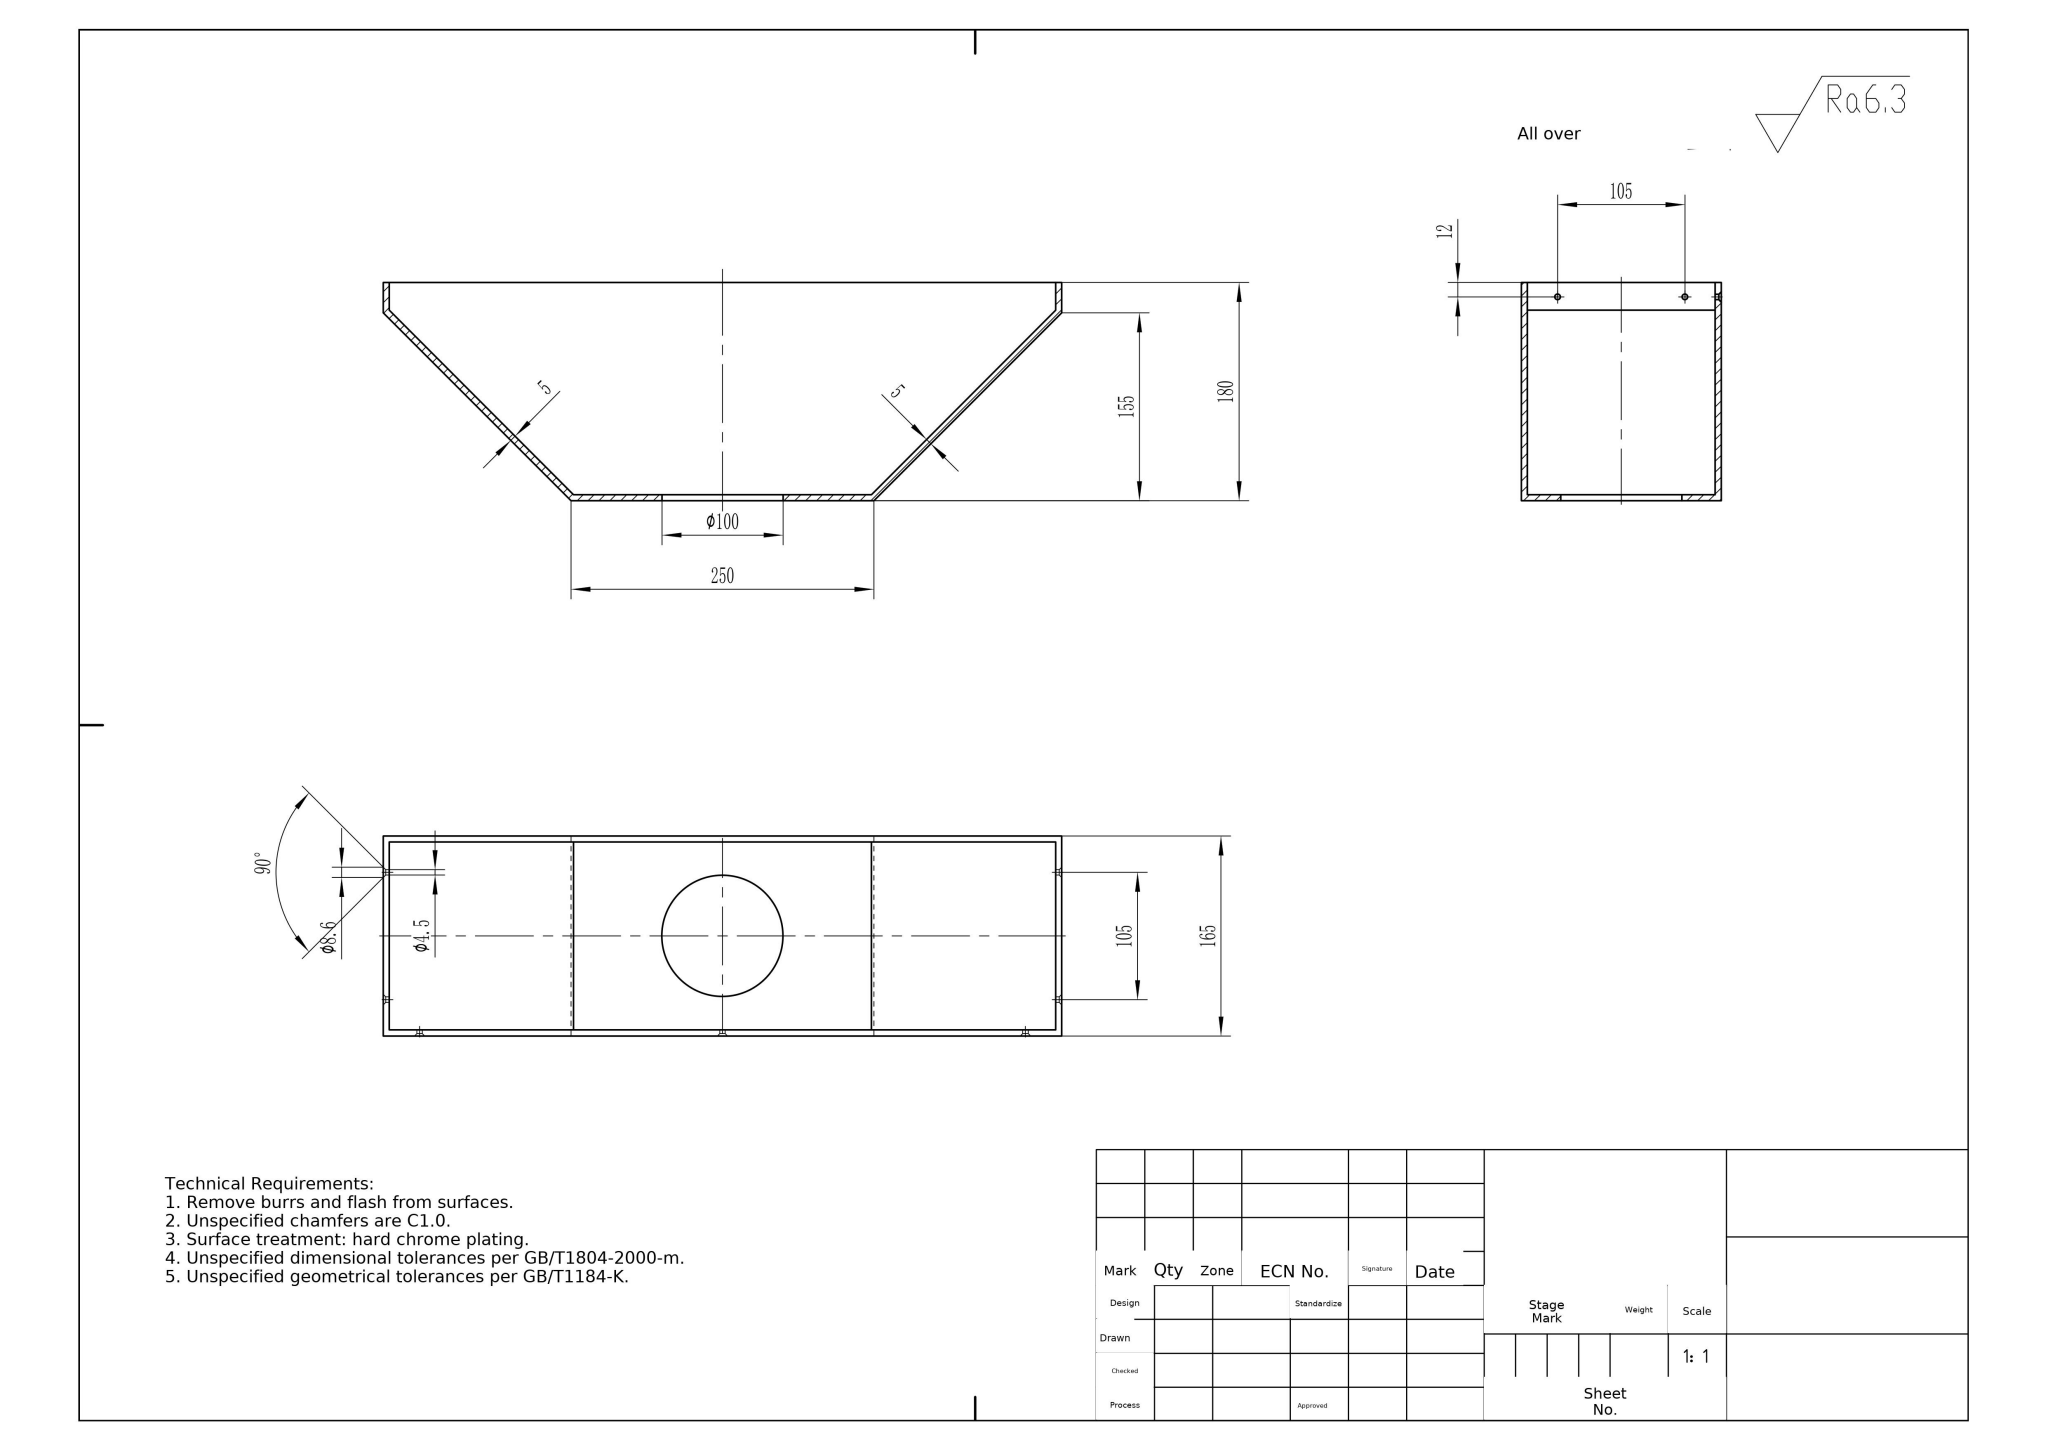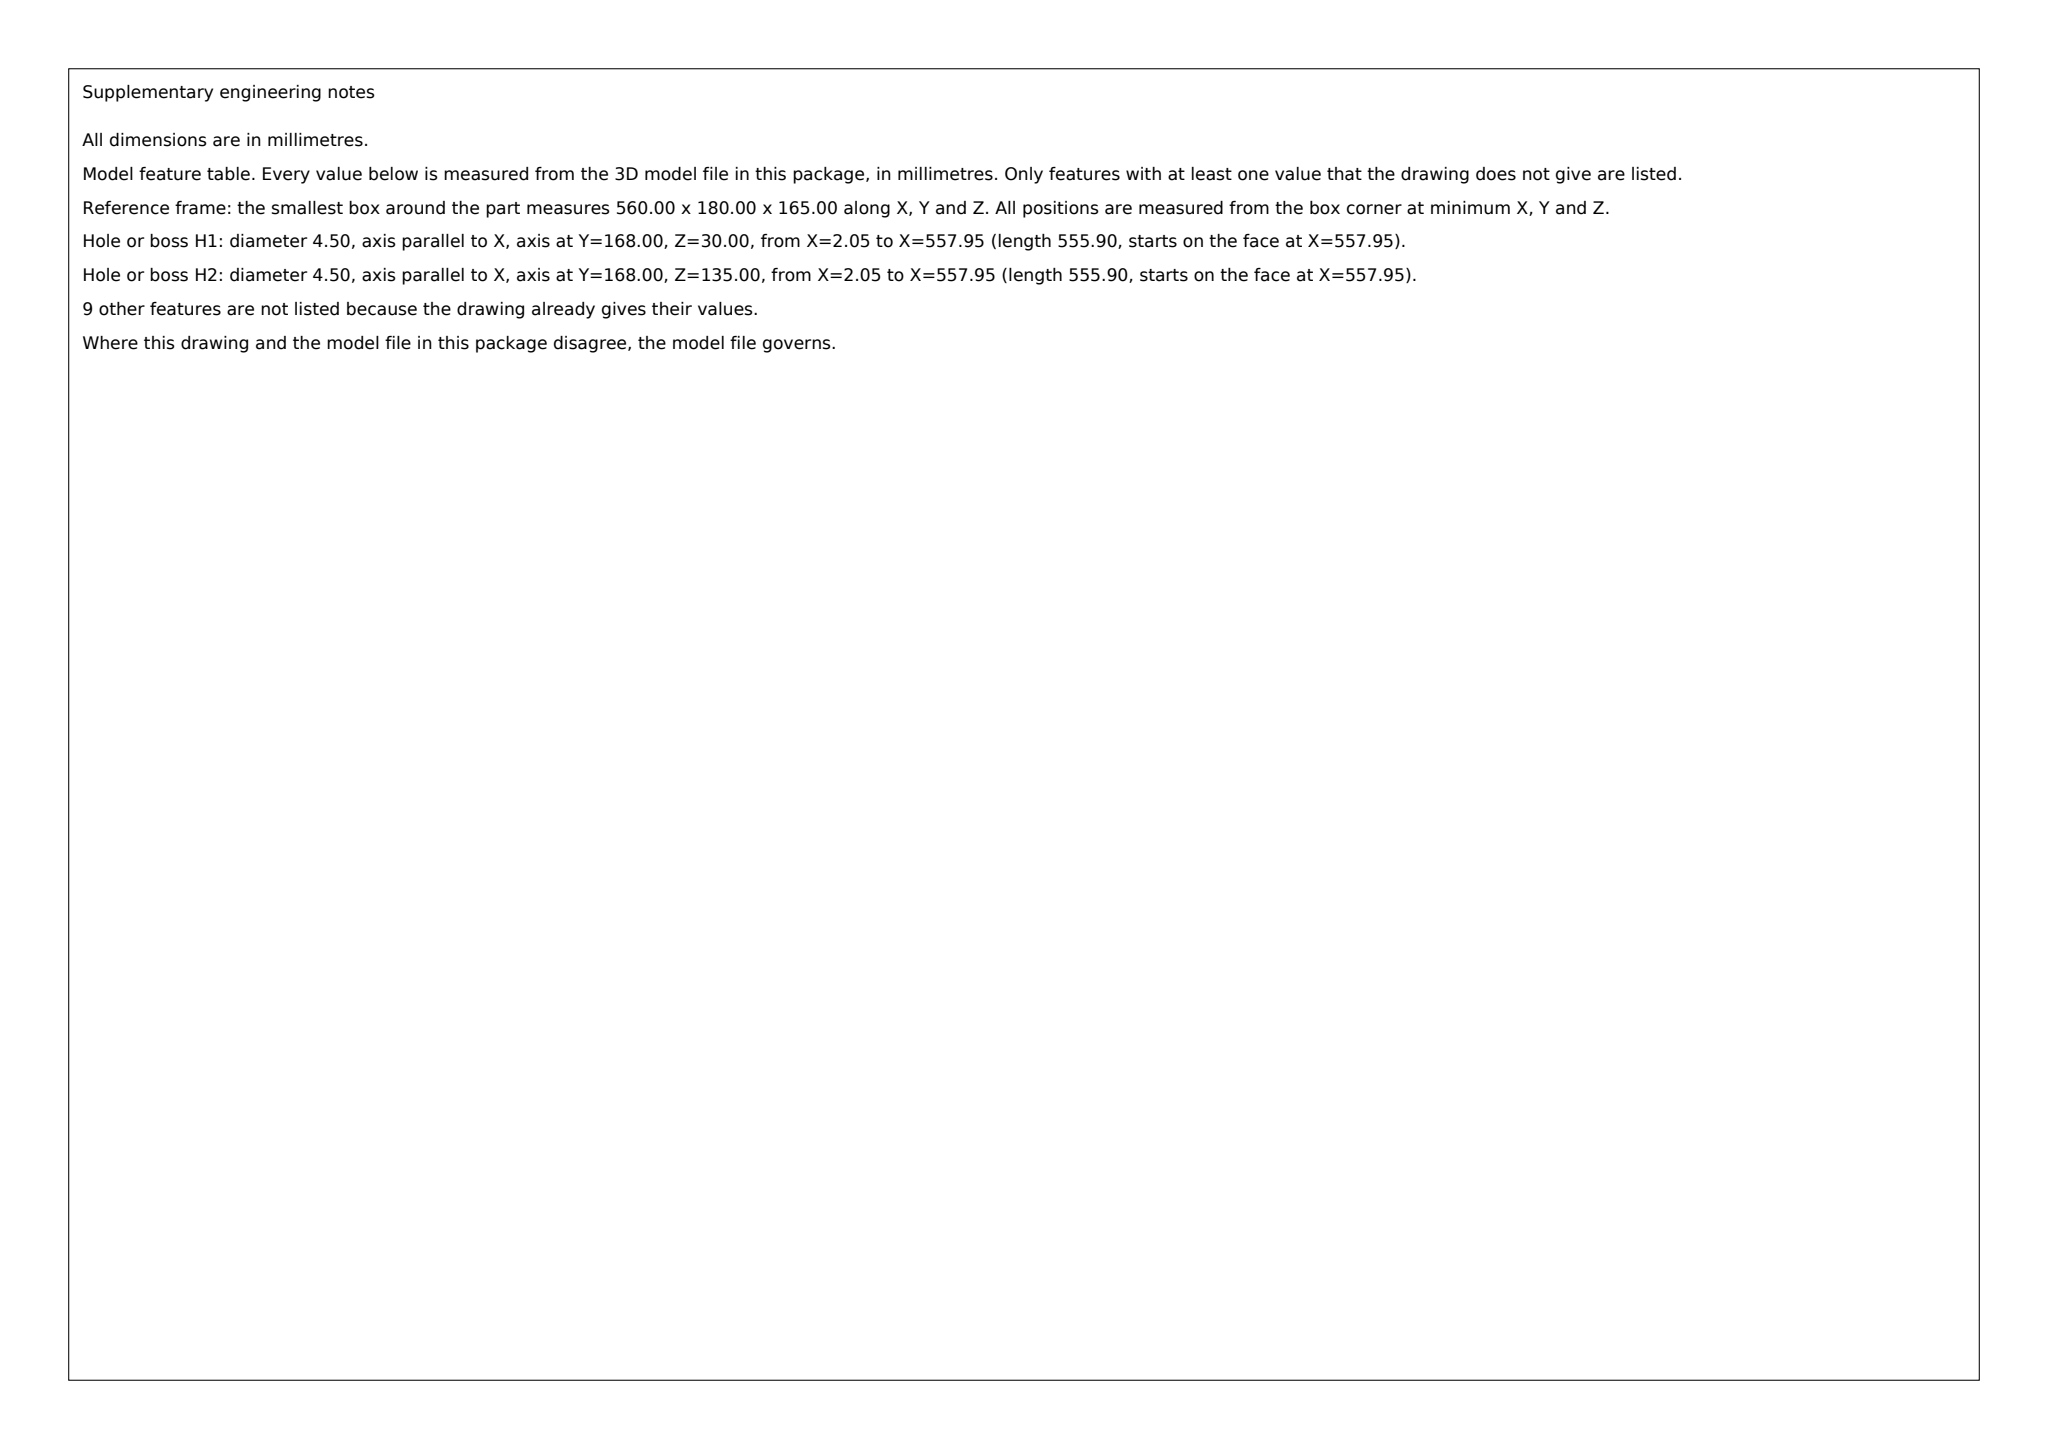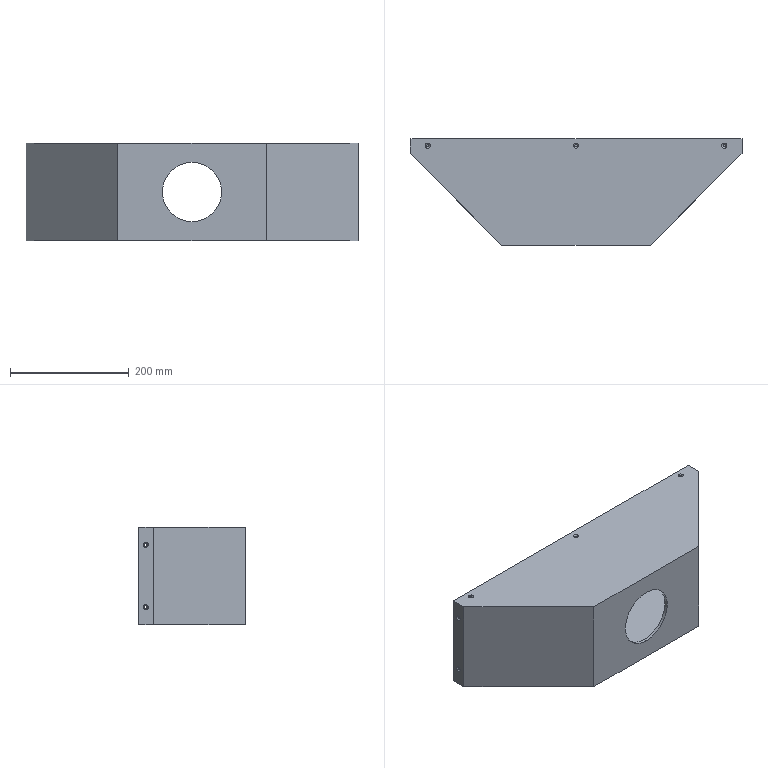Part | SolidWorks | mm | 1 solid | 45 faces | box 560 x 180 x 165 mm | volume 1293497 mm3 | cylinder 16 | plane 15 | cone 14 | commonest cylinder face diameters 4.5 x14 100 x2
build123d program:
from build123d import *

# Parameters (mm, degrees)
BOSS_EXTRUDE1_DEPTH                               = 82.5
SHELL1_T                                          = -5
SKETCH2_R                                         = 50
CUT_EXTRUDE1_DEPTH                                = 341.34
HOLE_SIZE_ACCORDING_TO_PHILLIPS_RAISE_D           = 4.5
HOLE_SIZE_ACCORDING_TO_PHILLIPS_RAISE_DEPTH       = 5.001
HOLE_SIZE_ACCORDING_TO_PHILLIPS_RAISE_CSINK_D     = 8.6
HOLE_SIZE_ACCORDING_TO_PHILLIPS_RAISE_CSINK_ANGLE = 90
MIRROR2_COPY_1_D                                  = 4.5
MIRROR2_COPY_1_DEPTH                              = 5.001
MIRROR2_COPY_1_CSINK_D                            = 8.6
MIRROR2_COPY_1_CSINK_ANGLE                        = 90
HOLE_SIZE_ACCORDING_TO_PHILLIPS_R_2_D             = 4.5
HOLE_SIZE_ACCORDING_TO_PHILLIPS_R_2_DEPTH         = 5
HOLE_SIZE_ACCORDING_TO_PHILLIPS_R_2_CSINK_D       = 8.6
HOLE_SIZE_ACCORDING_TO_PHILLIPS_R_2_CSINK_ANGLE   = 90


with BuildPart() as part:
    # Sketch1 → Boss-Extrude1 (new, symmetric)
    with BuildSketch(Plane.XY):
        Polygon((125, 0), (-125, 0), (-280, 155), (-280, 180), (280, 180), (280, 155), align=None)
    extrude(amount=BOSS_EXTRUDE1_DEPTH, both=True)

    # Shell1
    shell1_openings = [part.faces().sort_by_distance(p)[0] for p in [
        (0, 180, 0),
    ]]
    offset(amount=SHELL1_T, openings=shell1_openings, kind=Kind.INTERSECTION)

    # Sketch2 → Cut-Extrude1 (cut, through all)
    with BuildSketch(Plane(origin=(0, 5, 0), x_dir=(1, 0, 0), z_dir=(0, 1, 0))):
        with Locations(Location((0, 0, 0), (0, 0, 270))):
            Circle(SKETCH2_R)
    extrude(amount=-CUT_EXTRUDE1_DEPTH, mode=Mode.SUBTRACT)

    # Hole Size _ according to Phillips_ Raise
    with Locations(Plane.ZY.offset(280)):
        with Locations((-52.5, 168)):
            hole_size_according_to_phillips_raise = CounterSinkHole(HOLE_SIZE_ACCORDING_TO_PHILLIPS_RAISE_D / 2, HOLE_SIZE_ACCORDING_TO_PHILLIPS_RAISE_CSINK_D / 2, depth=HOLE_SIZE_ACCORDING_TO_PHILLIPS_RAISE_DEPTH, counter_sink_angle=HOLE_SIZE_ACCORDING_TO_PHILLIPS_RAISE_CSINK_ANGLE)

    # Mirror1: Hole Size _ according to Phillips_ Raise across plane
    add(hole_size_according_to_phillips_raise.mirror(Plane.XY), mode=Mode.SUBTRACT)

    # Mirror2: Hole Size _ according to Phillips_ Raise across plane
    add(hole_size_according_to_phillips_raise.mirror(Plane(origin=(0, 0, 0), x_dir=(0, 0, 1), z_dir=(1, 0, 0))), mode=Mode.SUBTRACT)

    # Mirror2 copy 1
    with Locations(Plane(origin=(280, 0, 0), x_dir=(0, 0, -1), z_dir=(1, 0, 0))):
        with Locations((-52.5, 168)):
            CounterSinkHole(MIRROR2_COPY_1_D / 2, MIRROR2_COPY_1_CSINK_D / 2, depth=MIRROR2_COPY_1_DEPTH, counter_sink_angle=MIRROR2_COPY_1_CSINK_ANGLE)

    # Hole Size _ according to Phillips_ R 2
    with Locations(Plane.XY.offset(82.5)):
        with Locations((-250, 168), (0, 168), (250, 168)):
            CounterSinkHole(HOLE_SIZE_ACCORDING_TO_PHILLIPS_R_2_D / 2, HOLE_SIZE_ACCORDING_TO_PHILLIPS_R_2_CSINK_D / 2, depth=HOLE_SIZE_ACCORDING_TO_PHILLIPS_R_2_DEPTH, counter_sink_angle=HOLE_SIZE_ACCORDING_TO_PHILLIPS_R_2_CSINK_ANGLE)


solid = part.part